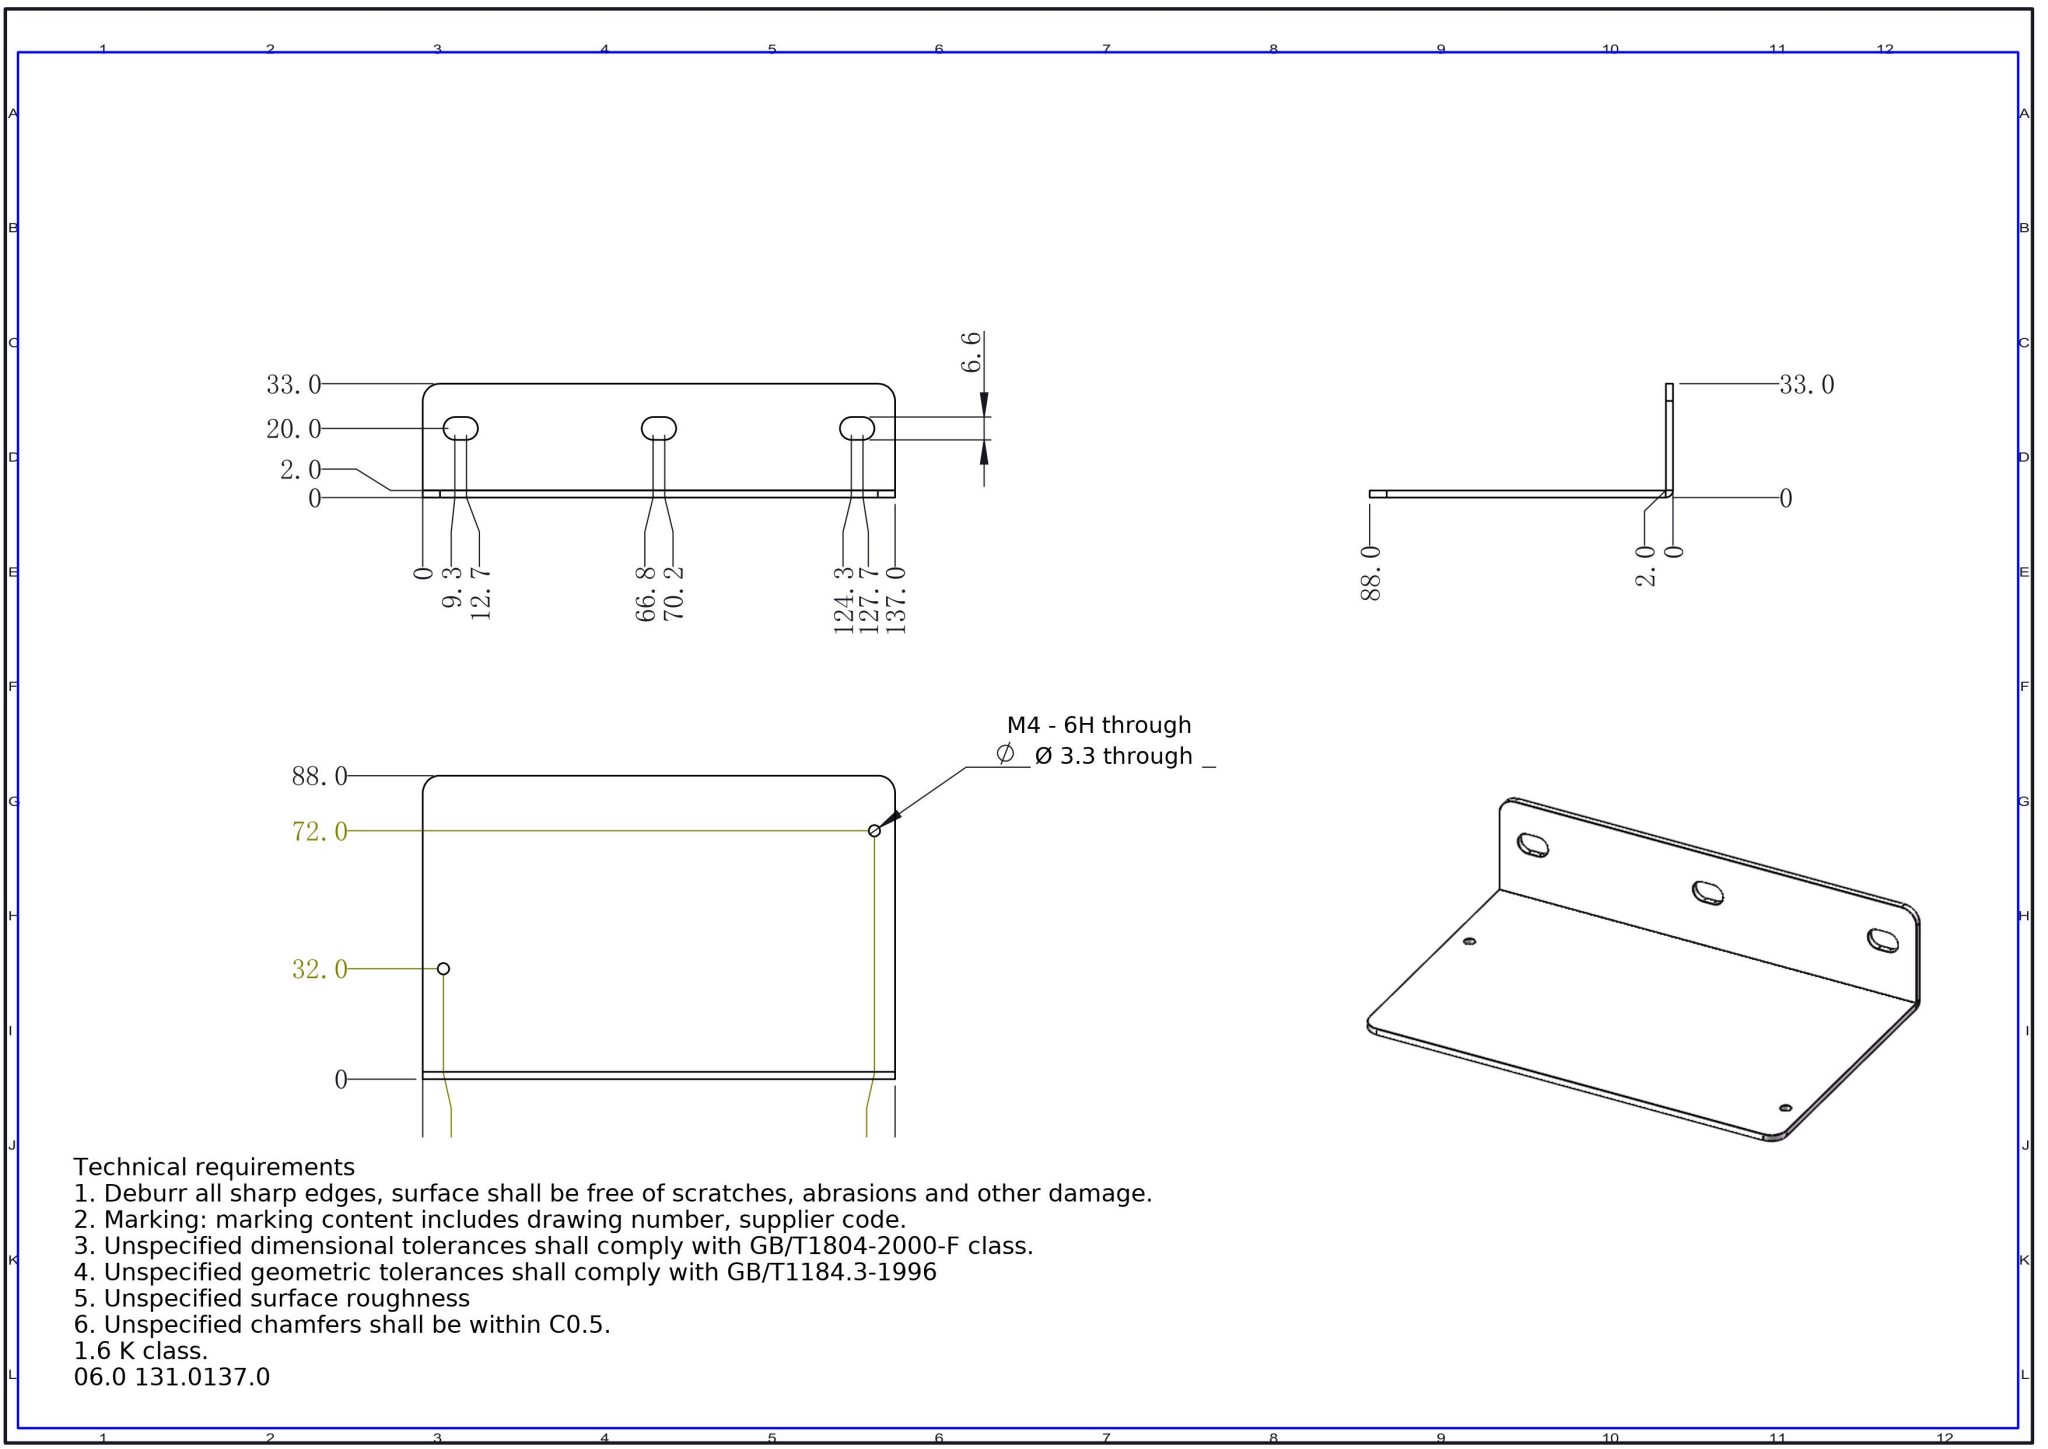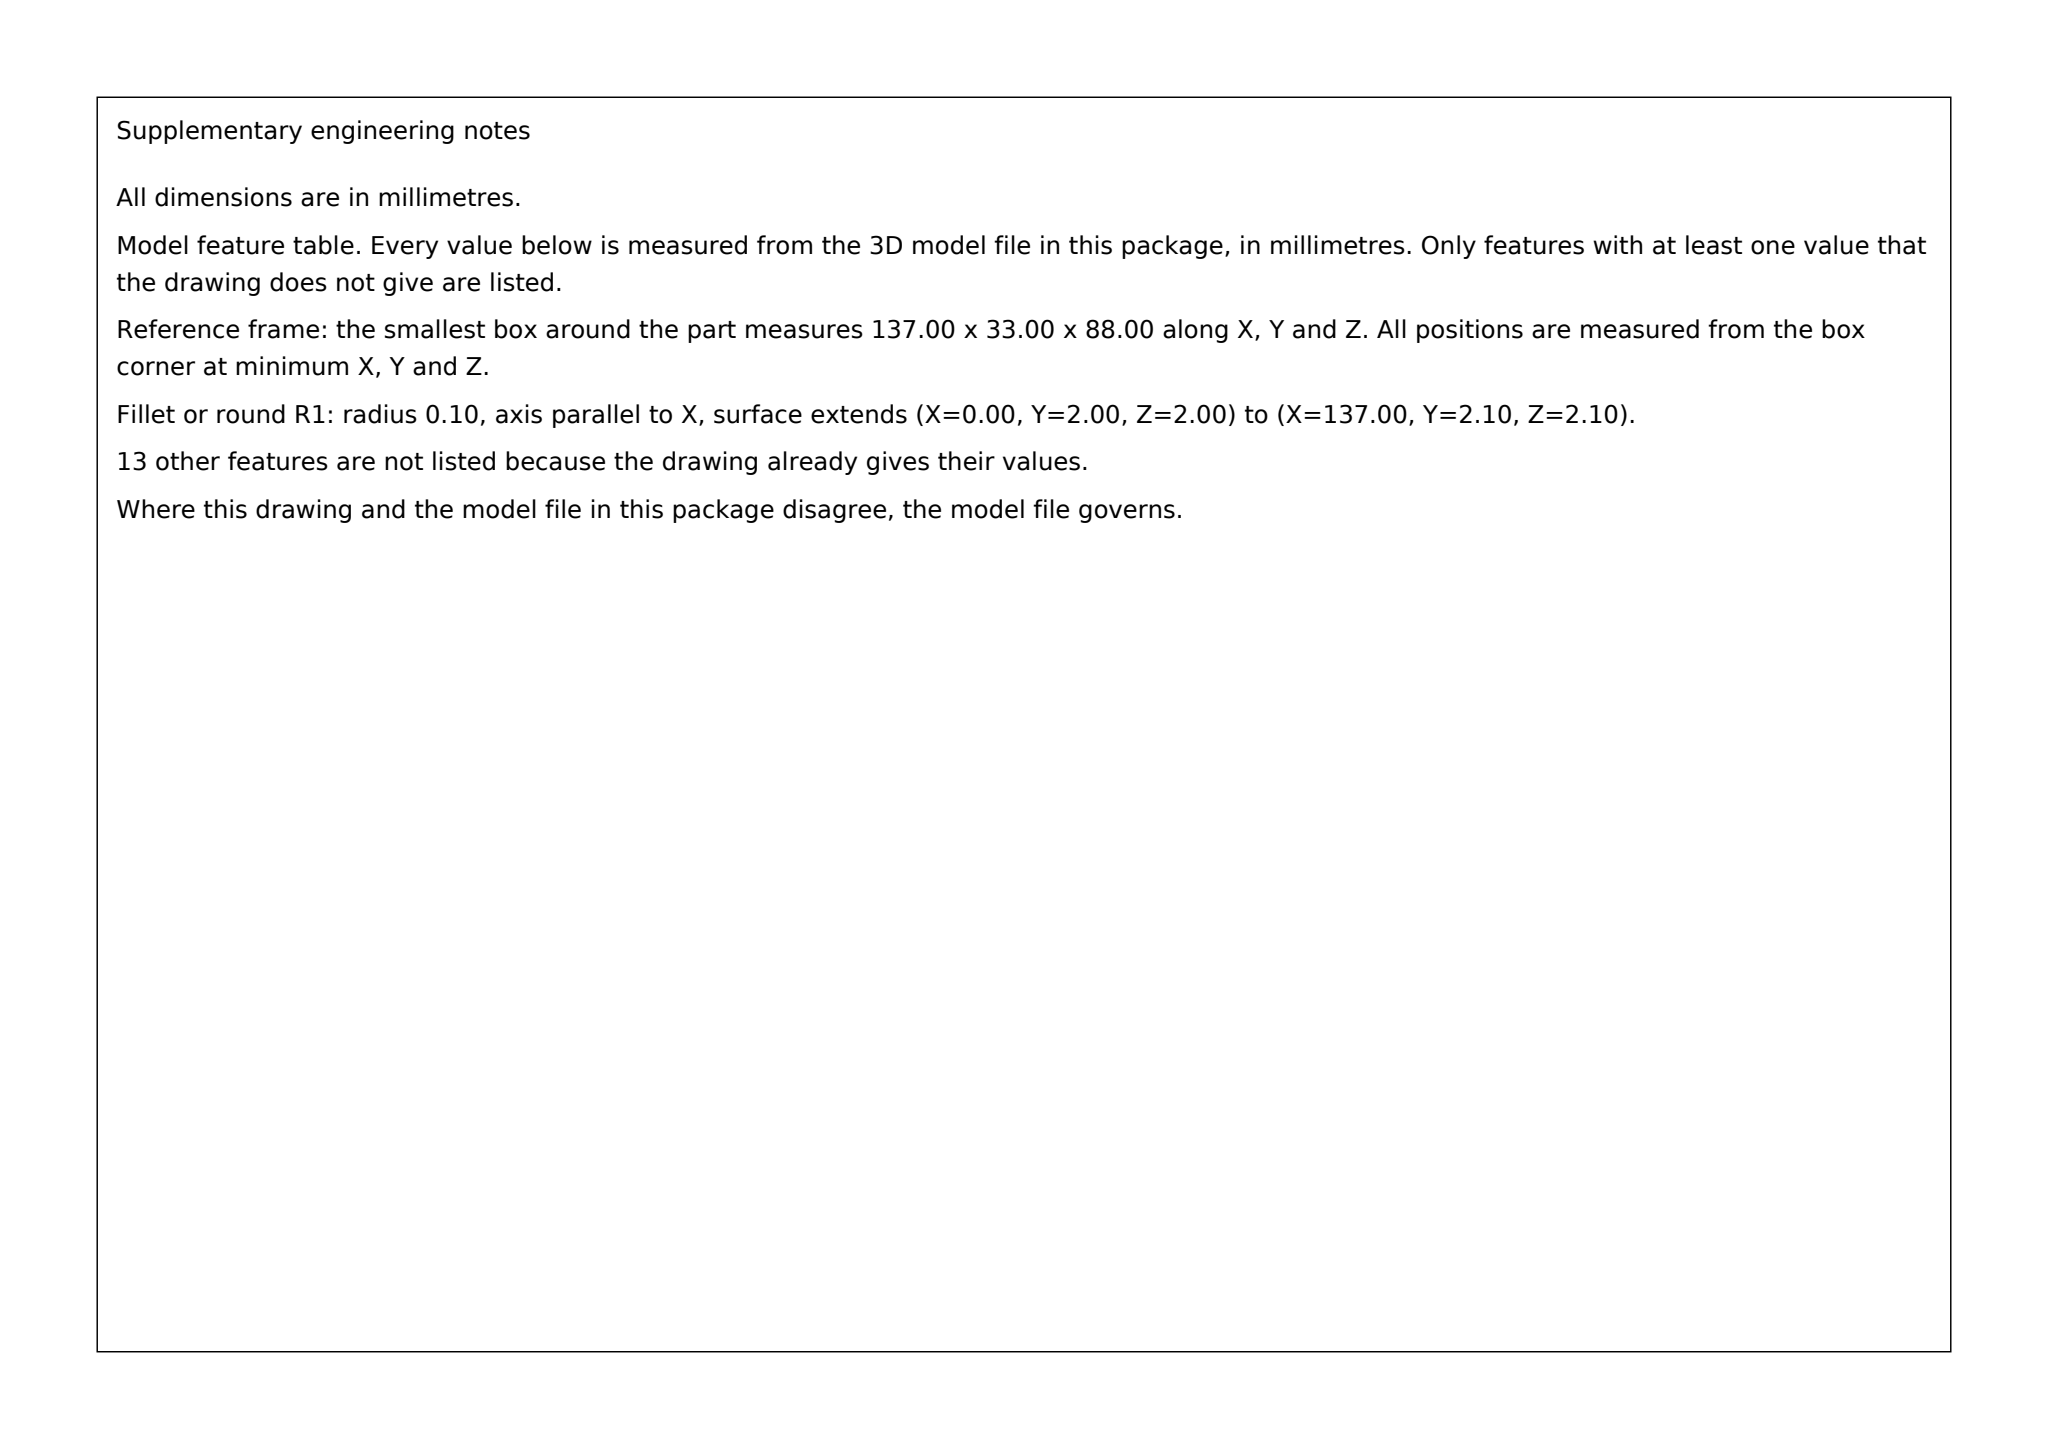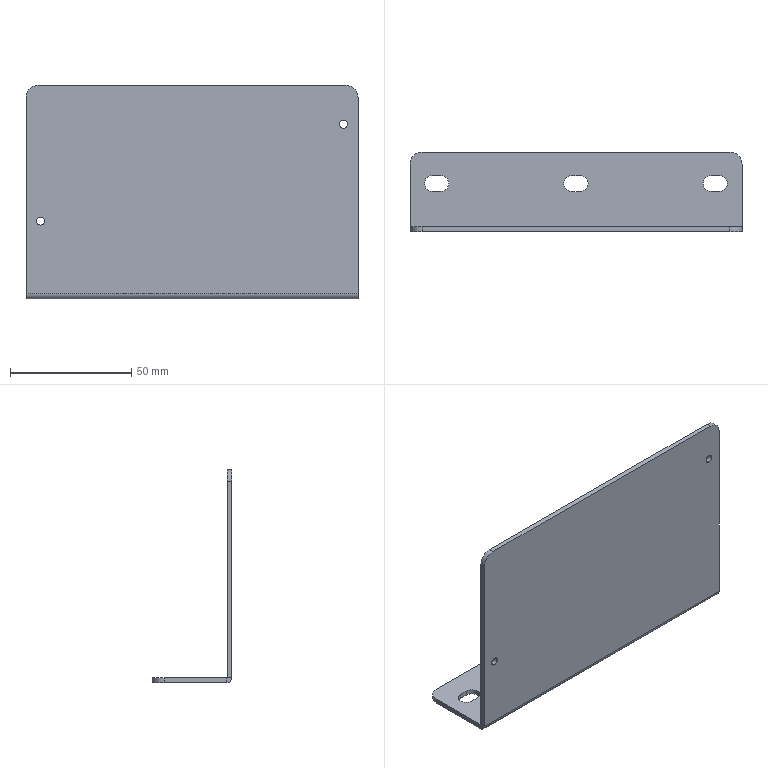Part | SolidWorks | mm | 1 solid | 37 faces | box 137 x 33 x 88 mm | volume 32060 mm3 | cylinder 19 | plane 18 | commonest cylinder face diameters 6.6 x9 3.3 x4 10 x4 4.2 x1 0.2 x1